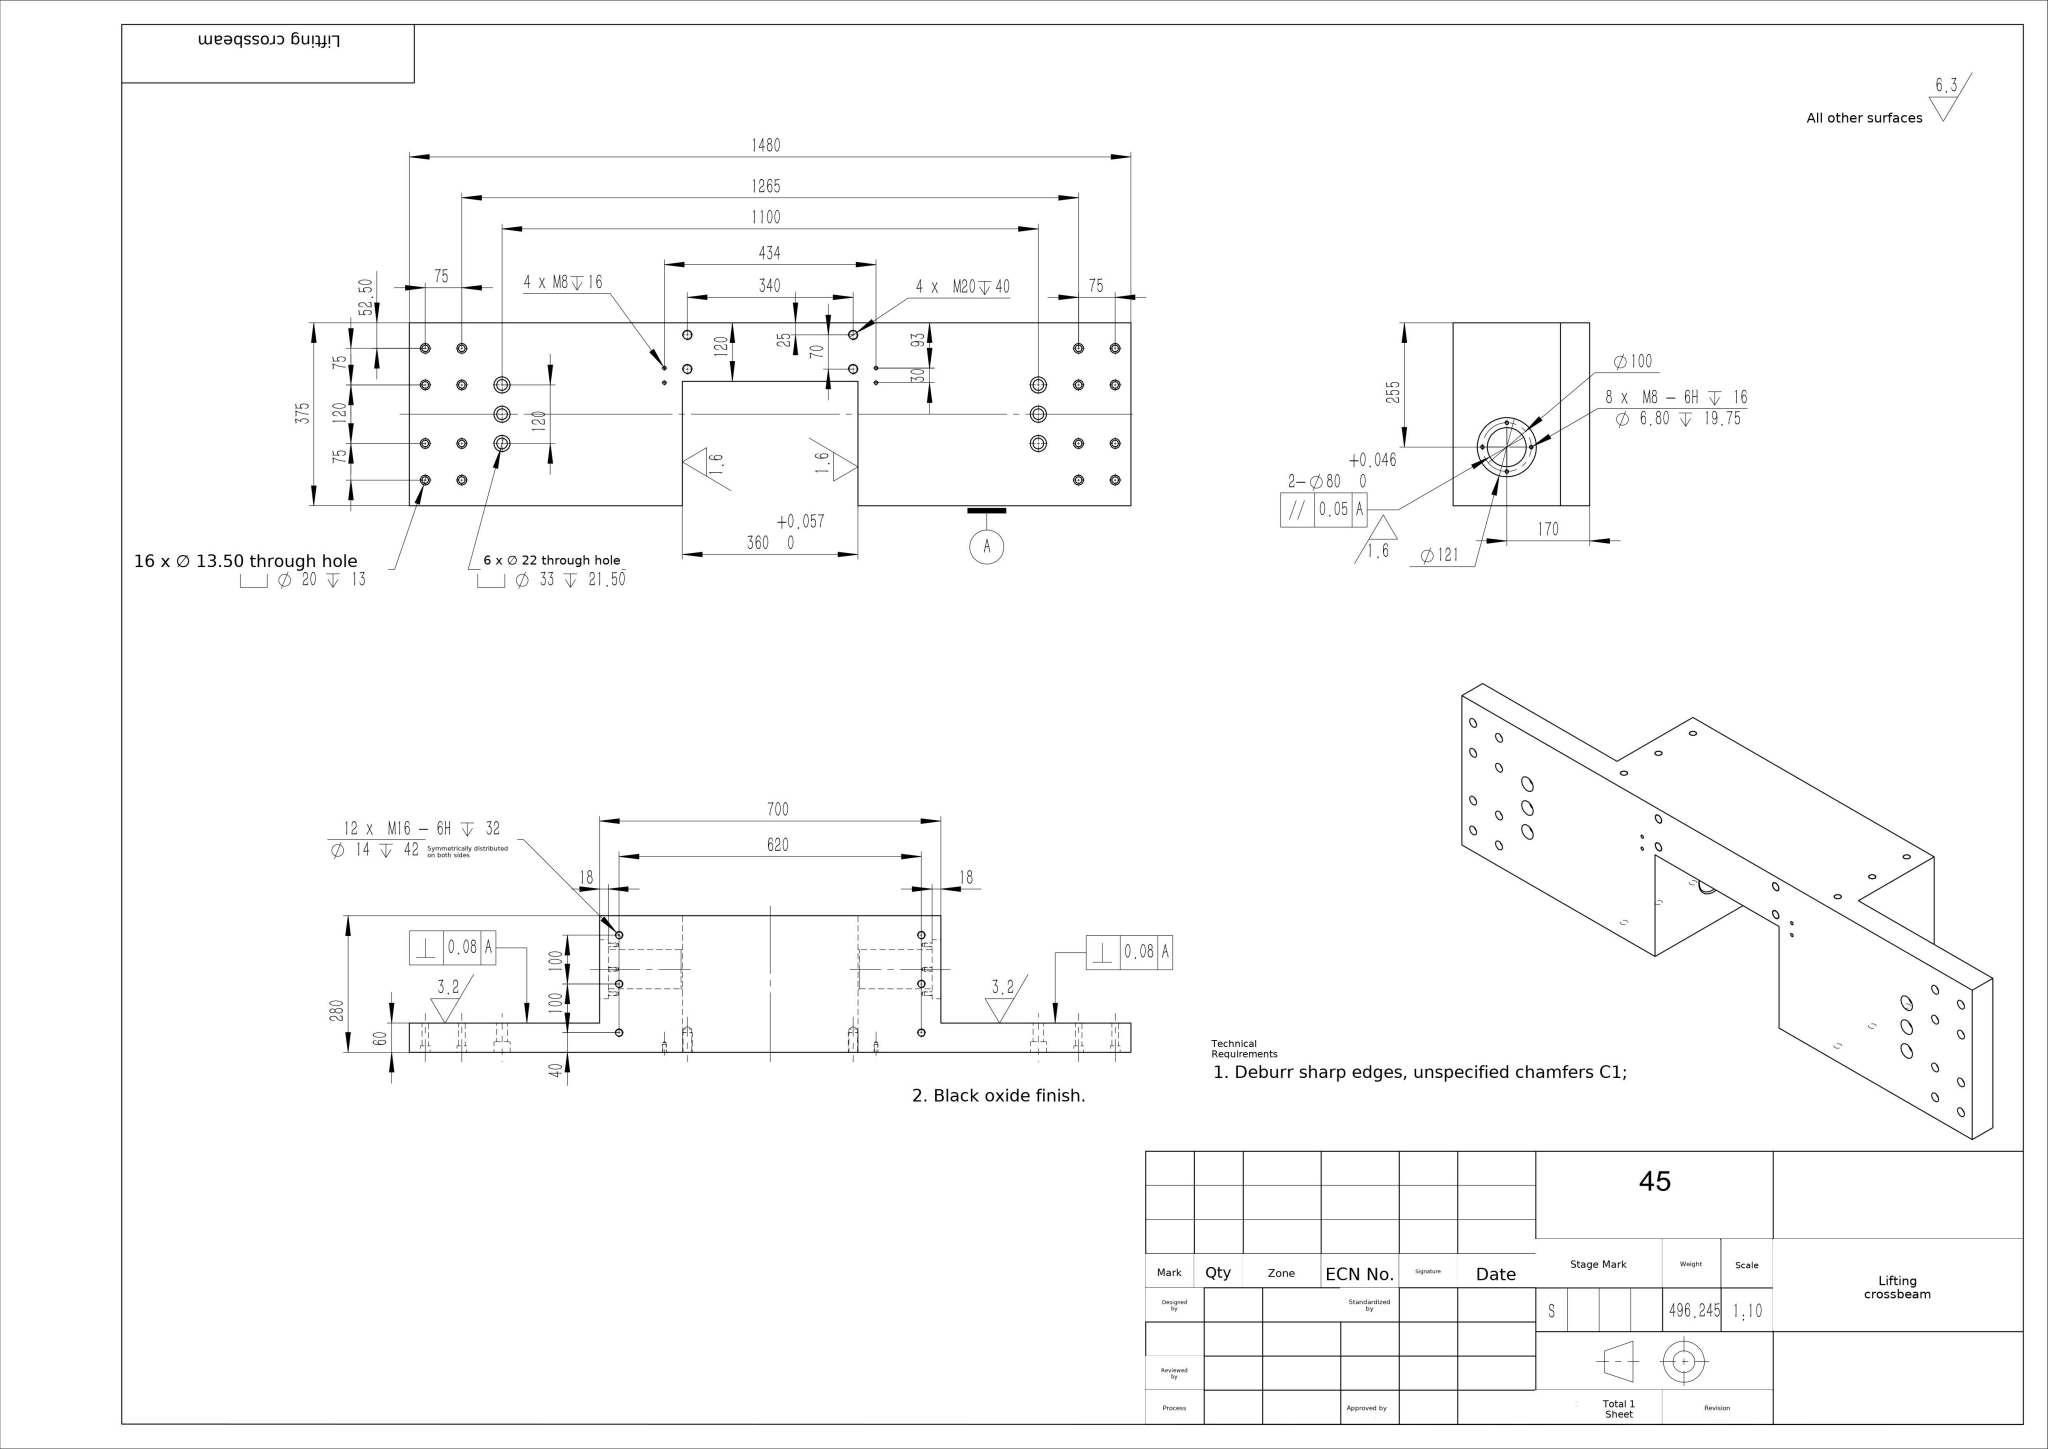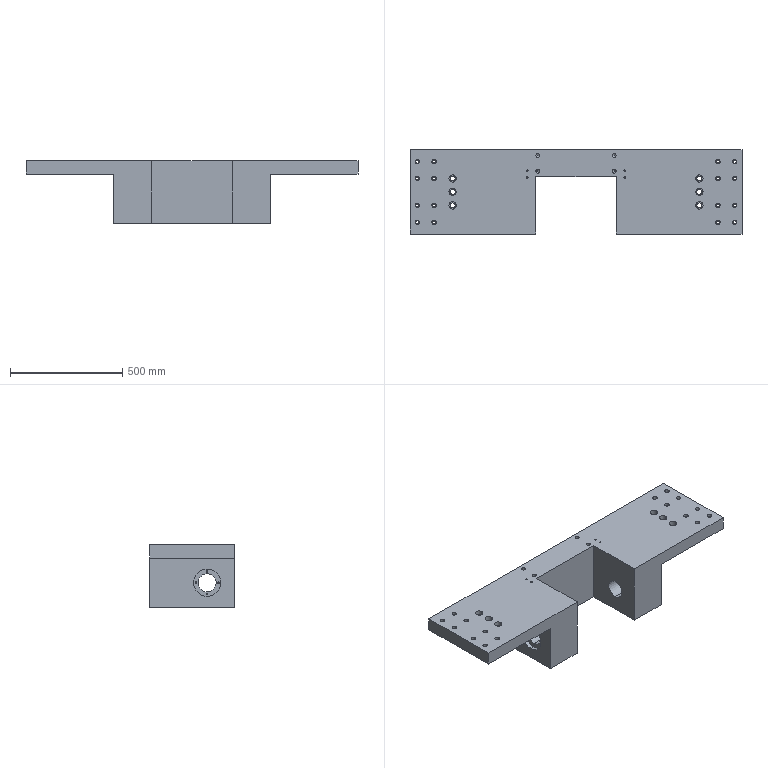Part | SolidWorks | mm | 1 solid | 222 faces | box 1480 x 375 x 280 mm | volume 62931284 mm3 | cylinder 140 | cone 44 | plane 38 | commonest cylinder face diameters 20 x32 13.5 x32 6.8 x24 14 x12 33 x12 22 x12 17.5 x8 80 x4
build123d program:
from build123d import *

# Parameters (mm, degrees)
BOSS_EXTRUDE1_DEPTH                               = 280
SKETCH2_W                                         = 390
SKETCH2_H                                         = 220
CUT_EXTRUDE1_DEPTH                                = 1553.232
HOLE_SIZE_ACCORDING_TO_HEXAGON_SOCKET_D           = 13.5
HOLE_SIZE_ACCORDING_TO_HEXAGON_SOCKET_CBORE_D     = 20
HOLE_SIZE_ACCORDING_TO_HEXAGON_SOCKET_CBORE_DEPTH = 13
HOLE_SIZE_ACCORDING_TO_HEXAGON_SO_2_D             = 22
HOLE_SIZE_ACCORDING_TO_HEXAGON_SO_2_CBORE_D       = 33
HOLE_SIZE_ACCORDING_TO_HEXAGON_SO_2_CBORE_DEPTH   = 21.5
M8_TAPPED_HOLE1_D                                 = 6.8
M8_TAPPED_HOLE1_DEPTH                             = 22.25
M8_TAPPED_HOLE1_TIP                               = 2.043
M20_TAPPED_HOLE1_D                                = 17.5
M20_TAPPED_HOLE1_DEPTH                            = 52.5
M20_TAPPED_HOLE1_TIP                              = 5.258
M16_TAPPED_HOLE1_D                                = 14
M16_TAPPED_HOLE1_DEPTH                            = 42
M16_TAPPED_HOLE1_TIP                              = 4.206
SKETCH13_R                                        = 60.5
CUT_EXTRUDE2_DEPTH                                = 18
CUT_EXTRUDE3_REACH                                = 1171.705
SKETCH14_R                                        = 40
M8_TAPPED_HOLE2_AT_2_COUNT                        = 2
M8_TAPPED_HOLE2_AT_2_PITCH                        = 70.711
M8_TAPPED_HOLE2_AT_3_COUNT                        = 2
M8_TAPPED_HOLE2_AT_3_PITCH                        = 100
M8_TAPPED_HOLE2_AT_4_COUNT                        = 2
M8_TAPPED_HOLE2_AT_4_PITCH                        = 70.711


with BuildPart() as part:
    # Sketch1 → Boss-Extrude1 (new body)
    with BuildSketch(Plane.XY):
        Polygon((0, 0), (1480, 0), (1480, -375), (920, -375), (920, -120), (560, -120), (560, -375), (0, -375), align=None)
    extrude(amount=BOSS_EXTRUDE1_DEPTH)

    # Sketch2 → Cut-Extrude1 (cut, through all)
    with BuildSketch(Plane(origin=(0, 0, 0), x_dir=(1, 0, 0), z_dir=(0, 1, 0))):
        with Locations((195, -110)):
            Rectangle(SKETCH2_W, SKETCH2_H)
        with Locations((1285, -110)):
            Rectangle(SKETCH2_W, SKETCH2_H)
    extrude(amount=-CUT_EXTRUDE1_DEPTH, mode=Mode.SUBTRACT)

    # Hole Size _ according to_ Hexagon Socket (through all)
    with Locations(Plane.XY.offset(280)):
        with Locations((32.5, -52.5), (107.5, -52.5), (107.5, -127.5), (32.5, -127.5), (32.5, -247.5), (107.5, -247.5), (107.5, -322.5), (32.5, -322.5), (1447.5, -322.5), (1372.5, -322.5), (1372.5, -247.5), (1447.5, -247.5), (1447.5, -127.5), (1372.5, -127.5), (1372.5, -52.5), (1447.5, -52.5)):
            CounterBoreHole(HOLE_SIZE_ACCORDING_TO_HEXAGON_SOCKET_D / 2, HOLE_SIZE_ACCORDING_TO_HEXAGON_SOCKET_CBORE_D / 2, HOLE_SIZE_ACCORDING_TO_HEXAGON_SOCKET_CBORE_DEPTH)

    # Hole Size _ according to_ Hexagon So 2 (through all)
    with Locations(Plane.XY.offset(280)):
        with Locations((190, -127.5), (190, -187.5), (190, -247.5), (1290, -247.5), (1290, -187.5), (1290, -127.5)):
            CounterBoreHole(HOLE_SIZE_ACCORDING_TO_HEXAGON_SO_2_D / 2, HOLE_SIZE_ACCORDING_TO_HEXAGON_SO_2_CBORE_D / 2, HOLE_SIZE_ACCORDING_TO_HEXAGON_SO_2_CBORE_DEPTH)

    # M8 Tapped Hole1
    with Locations(Plane.XY.offset(280)):
        with Locations((523, -123), (523, -93), (957, -123), (957, -93)):
            Hole(M8_TAPPED_HOLE1_D / 2, depth=M8_TAPPED_HOLE1_DEPTH)
            with Locations((0, 0, -(M8_TAPPED_HOLE1_DEPTH + M8_TAPPED_HOLE1_TIP / 2))):  # 118° drill point
                Cone(0, M8_TAPPED_HOLE1_D / 2, M8_TAPPED_HOLE1_TIP, mode=Mode.SUBTRACT)

    # M20 Tapped Hole1
    with Locations(Plane.XY.offset(280)):
        with Locations((570, -25), (570, -95), (910, -95), (910, -25)):
            Hole(M20_TAPPED_HOLE1_D / 2, depth=M20_TAPPED_HOLE1_DEPTH)
            with Locations((0, 0, -(M20_TAPPED_HOLE1_DEPTH + M20_TAPPED_HOLE1_TIP / 2))):  # 118° drill point
                Cone(0, M20_TAPPED_HOLE1_D / 2, M20_TAPPED_HOLE1_TIP, mode=Mode.SUBTRACT)

    # M16 Tapped Hole1
    with Locations(Plane(origin=(0, 0, 0), x_dir=(1, 0, 0), z_dir=(0, 1, 0))):
        with Locations((430, -40), (430, -140), (430, -240), (1050, -40), (1050, -140), (1050, -240)):
            Hole(M16_TAPPED_HOLE1_D / 2, depth=M16_TAPPED_HOLE1_DEPTH)
            with Locations((0, 0, -(M16_TAPPED_HOLE1_DEPTH + M16_TAPPED_HOLE1_TIP / 2))):  # 118° drill point
                Cone(0, M16_TAPPED_HOLE1_D / 2, M16_TAPPED_HOLE1_TIP, mode=Mode.SUBTRACT)

    # Sketch13 → Cut-Extrude2 (cut)
    with BuildSketch(Plane.ZY.offset(-390)):
        with Locations((110, -255)):
            Circle(SKETCH13_R)
    cut_extrude2 = extrude(amount=-CUT_EXTRUDE2_DEPTH, mode=Mode.SUBTRACT)

    # Sketch14 → Cut-Extrude3 (cut, up to next)
    with BuildSketch(Plane.ZY.offset(-408), mode=Mode.PRIVATE) as cut_extrude3_sk1:
        with Locations((110, -255)):
            Circle(SKETCH14_R)
    cut_extrude3_tool1 = extrude(cut_extrude3_sk1.sketch, amount=-CUT_EXTRUDE3_REACH, mode=Mode.PRIVATE) & part.part
    cut_extrude3 = cut_extrude3_tool1.solids().sort_by_distance((408, -255, 110))[0]
    add(cut_extrude3, mode=Mode.SUBTRACT)

    # Sketch16 → M8 Tapped Hole2 (revolve, cut)
    with BuildSketch(Plane(origin=(408, -205, 110), x_dir=(0, 0, 1), z_dir=(0, 1, 0))):
        Polygon((0, 0), (0, 21.793), (3.4, 19.75), (3.4, 0), align=None)
    m8_tapped_hole2 = revolve(axis=Axis((401.65, -205, 110), (1, 0, 0)), mode=Mode.SUBTRACT)

    # M8 Tapped Hole2 at 2: M8 Tapped Hole2 ×2
    with Locations(*[Vector(0, -0.7071, 0.7071) * (i * M8_TAPPED_HOLE2_AT_2_PITCH) for i in range(1, M8_TAPPED_HOLE2_AT_2_COUNT)]):
        add(m8_tapped_hole2, mode=Mode.SUBTRACT)

    # M8 Tapped Hole2 at 3: M8 Tapped Hole2 ×2
    with Locations(*[(0, -i * M8_TAPPED_HOLE2_AT_3_PITCH, 0) for i in range(1, M8_TAPPED_HOLE2_AT_3_COUNT)]):
        add(m8_tapped_hole2, mode=Mode.SUBTRACT)

    # M8 Tapped Hole2 at 4: M8 Tapped Hole2 ×2
    with Locations(*[Vector(0, -0.7071, -0.7071) * (i * M8_TAPPED_HOLE2_AT_4_PITCH) for i in range(1, M8_TAPPED_HOLE2_AT_4_COUNT)]):
        add(m8_tapped_hole2, mode=Mode.SUBTRACT)

    # Mirror1: Cut-Extrude2, Cut-Extrude3, M8 Tapped Hole2 across plane
    add(cut_extrude2.mirror(Plane(origin=(740, 0, 0), x_dir=(0, 0, 1), z_dir=(1, 0, 0))), mode=Mode.SUBTRACT)
    add(cut_extrude3.mirror(Plane(origin=(740, 0, 0), x_dir=(0, 0, 1), z_dir=(1, 0, 0))), mode=Mode.SUBTRACT)
    add(m8_tapped_hole2.mirror(Plane(origin=(740, 0, 0), x_dir=(0, 0, 1), z_dir=(1, 0, 0))), mode=Mode.SUBTRACT)

    # Mirror1 copy 1 sketch → Mirror1 copy 1 (revolve, cut)
    with BuildSketch(Plane(origin=(1072, -255, 160), x_dir=(0, 0, 1), z_dir=(0, 1, 0))):
        Polygon((0, 0), (0, -21.793), (3.4, -19.75), (3.4, 0), align=None)
    revolve(axis=Axis((1078.35, -255, 160), (1, 0, 0)), mode=Mode.SUBTRACT)

    # Mirror1 copy 2 sketch → Mirror1 copy 2 (revolve, cut)
    with BuildSketch(Plane(origin=(1072, -305, 110), x_dir=(0, 0, 1), z_dir=(0, 1, 0))):
        Polygon((0, 0), (0, -21.793), (3.4, -19.75), (3.4, 0), align=None)
    revolve(axis=Axis((1078.35, -305, 110), (1, 0, 0)), mode=Mode.SUBTRACT)

    # Mirror1 copy 3 sketch → Mirror1 copy 3 (revolve, cut)
    with BuildSketch(Plane(origin=(1072, -255, 60), x_dir=(0, 0, 1), z_dir=(0, 1, 0))):
        Polygon((0, 0), (0, -21.793), (3.4, -19.75), (3.4, 0), align=None)
    revolve(axis=Axis((1078.35, -255, 60), (1, 0, 0)), mode=Mode.SUBTRACT)


solid = part.part